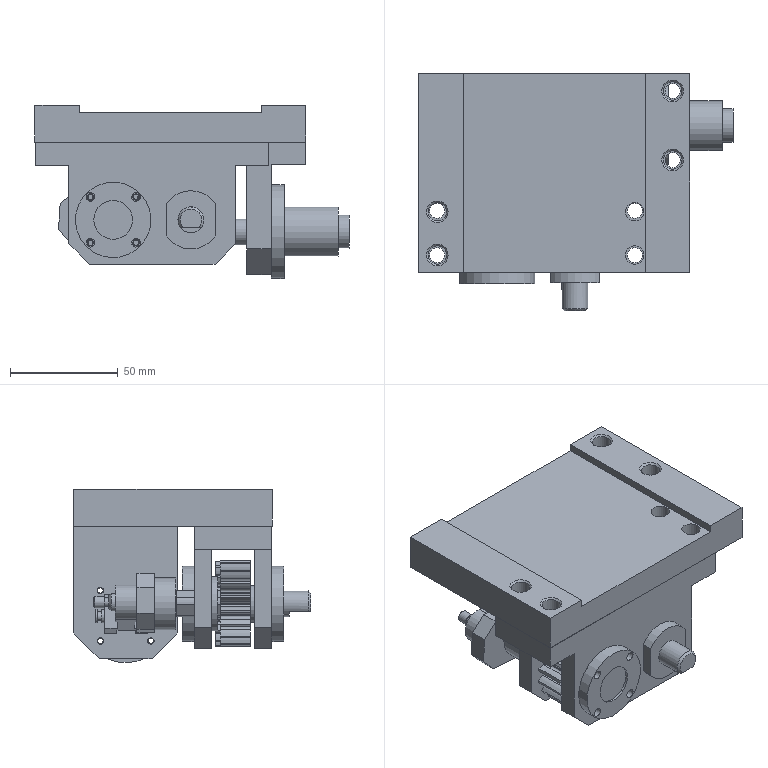Assembly | NX | mm | 16 component files | 16 solids | 549 faces | box 145.5 x 110 x 80.25 mm | volume 378526 mm3 | spline 182 | cylinder 153 | plane 150 | cone 63 | sphere 1 | commonest cylinder face diameters 30.9 x36 4 x14 12 x14 2.5 x12 18 x7 10 x7 8.5 x6 15 x6
Bill of materials:
unnamed part 1 | 1 |  | Stepped cylindrical shaft with a thin integral collar near one end, a larger-diameter section, a middle section with a flat face along it, and a smaller-diameter far end; both ends chamfered.
unnamed part 2 | 1 |  | Elongated link or lever with rounded ends. One end is a single lug with a larger through hole. The other end is a fork with two parallel lugs, a slot between them, and a smaller cross hole through both lugs. The middle bar is narrower than the ends.
unnamed part 3 | 2 |  | Spur gear with straight teeth, about 18 of them, a plain face on each side, and a central round bore with a single rectangular keyway.
unnamed part 4 | 1 |  | Flanged cylindrical hub: a circular flange with four through holes on a square pattern, a long cylindrical body on one side ending in a smaller pilot step, a short chamfered boss on the other side, and a central through bore.
unnamed part 5 | 1 |  | Bracket with a rectangular top plate carrying four through holes near its corners and two parallel walls hanging below it, giving an inverted-U end profile. The front wall has chamfered lower corners, two large through holes, and four small holes around one of the large holes.
unnamed part 6 | 1 |  | Rectangular plate with a shallow recess across most of its top face, leaving raised lands at both ends, and six through holes, several with chamfered or counterbored edges.
unnamed part 7 | 1 |  | L-shaped bracket: a horizontal top plate with two through holes and a vertical plate with chamfered lower corners. The vertical plate has a large central hole with internal steps or grooves and four small holes around it.
unnamed part 8 | 1 |  | Stepped cylindrical pin. A short end section has a transverse through hole and is followed by a narrow neck. Next come a larger cylindrical body, an integral collar, and a long smaller-diameter shaft with a chamfered end.
unnamed part 9 | 1 |  | Flanged bushing: a thin circular flange joined to a cylindrical sleeve, with a central through bore and a chamfered outer edge at the sleeve end.
unnamed part 10 | 1 |  | Stepped cylindrical shaft with a thin integral collar, a larger body section, and a long smaller section that has a flat (D-cut) along part of its length. The ends are chamfered.
unnamed part 11 | 2 |  | Circular flange with four through holes near its rim and a short cylindrical hub on one side. The hub has a narrow groove next to the flange and a chamfered end, with a bore opening at the hub end.
unnamed part 12 | 1 |  | Headed pin with a flat, chamfered disc head, a long plain cylindrical shank, and a circumferential groove near the far end that leaves a thin end lip.
unnamed part 13 | 1 |  | Flat plate shaped like a rectangle with chamfered (clipped) corners. One face carries a cylindrical boss with a central bore and a small radial cross hole. The opposite face carries a stepped cylindrical pin that ends in a smaller-diameter tip with a circumferential groove and chamfered ends. The pin axis appears offset from the boss axis.
unnamed part 14 | 1 |  | Flanged bushing with a through bore. The circular flange has two parallel flats cut on opposite sides. The cylindrical shank has a slightly reduced-diameter section next to the flange (a relief or step), and its free end has a chamfer.
Mates:
1. touch align | CLHKJG_01_Gear_Support 1 face | CLHKJG_01_Base 1 face
2. touch align | CLHKJG_01_Base 1 face | CLHKJG_01_Gear_Support 1 face
3. fix | CLHKJG_01_Base 1 component
4. touch align | CLHKJG_01_Gear_Support 1 face | CLHKJG_01_Base 1 face
5. touch align | CLHKJG_02_Seal_End_Cap 2 face | CLHKJG_01_Gear_Support 1 face
6. touch align | CLHKJG_02_Seal_End_Cap 2 face | CLHKJG_01_Gear_Support 1
7. touch align | CLHKJG_01_Gear_Support 1 face | CLHKJG_02_Seal_End_Cap 2 face
8. touch align | CLHKJG_05_Input_Shaft 1 face | CLHKJG_01_Gear_Support 1 face
9. touch align | CLHKJG_03_Output_Shaft 1 face | CLHKJG_01_Gear_Support 1 face
10. touch align | CLHKJG_06_Thread_Seal_Sleeve 1 face | CLHKJG_01_Gear_Support 1 face
11. touch align | CLHKJG_06_Thread_Seal_Sleeve 1 face | CLHKJG_01_Gear_Support 1 face
12. touch align | CLHKJG_04_Gear 2 face | CLHKJG_03_Output_Shaft 1 face
13. touch align | CLHKJG_08_Cylinder_Support 1 face | CLHKJG_01_Base 1 face
14. touch align | CLHKJG_01_Base 1 face | CLHKJG_08_Cylinder_Support 1 face
15. touch align | CLHKJG_08_Cylinder_Support 1 face | CLHKJG_01_Base 1 face
16. touch align | CLHKJG_09_Cylinder_Support 1 face | CLHKJG_08_Cylinder_Support 1 face
17. touch align | CLHKJG_09_Cylinder_Support 1 face | CLHKJG_08_Cylinder_Support 1 face
18. touch align | CLHKJG_09_Cylinder_Support 1 face | CLHKJG_08_Cylinder_Support 1 face
19. touch align | CLHKJG_10_Piston_Rod 1 face | CLHKJG_08_Cylinder_Support 1 face
20. touch align | CLHKJG_13_Eccentric_Sleeve 1 face | CLHKJG_01_Gear_Support 1 face
21. touch align | CLHKJG_14_Shaft_Sleeve 1 face | CLHKJG_01_Gear_Support 1 face
22. touch align | CLHKJG_14_Shaft_Sleeve 1 face | CLHKJG_01_Gear_Support 1 face
23. touch align | CLHKJG_05_Input_Shaft 1 face | CLHKJG_02_Seal_End_Cap 2 face
24. touch align | CLHKJG_12_Connecting_Rod 1 face | CLHKJG_13_Eccentric_Sleeve 1 face
25. touch align | CLHKJG_12_Connecting_Rod 1 face | CLHKJG_13_Eccentric_Sleeve 1 face
26. touch align | CLHKJG_10_Piston_Rod 1 face | CLHKJG_12_Connecting_Rod 1 face
27. touch align | CLHKJG_11_Pivot_Pin 1 face | CLHKJG_12_Connecting_Rod 1 face
28. touch align | CLHKJG_12_Connecting_Rod 1 face | CLHKJG_11_Pivot_Pin 1 face
29. touch align | CLHKJG_12_Connecting_Rod 1 face | CLHKJG_10_Piston_Rod 1 face
30. touch align | CLHKJG_05_Input_Shaft 1 face | CLHKJG_04_Gear 1 face
31. touch align | CLHKJG_02_Seal_End_Cap 1 face | CLHKJG_01_Gear_Support 1 face
32. touch align | CLHKJG_02_Seal_End_Cap 1 face | CLHKJG_01_Gear_Support 1 face
33. touch align | CLHKJG_02_Seal_End_Cap 1 face | CLHKJG_01_Gear_Support 1 face
34. touch align | CLHKJG_03_Output_Shaft 1 face | CLHKJG_02_Seal_End_Cap 1 face
35. touch align | CLHKJG_04_Gear 2 face | CLHKJG_03_Output_Shaft 1 face
36. touch align | CLHKJG_04_Gear 1 face | CLHKJG_05_Input_Shaft 1 face
37. touch align | CLHKJG_04_Gear 2 face | CLHKJG_04_Gear 1 face